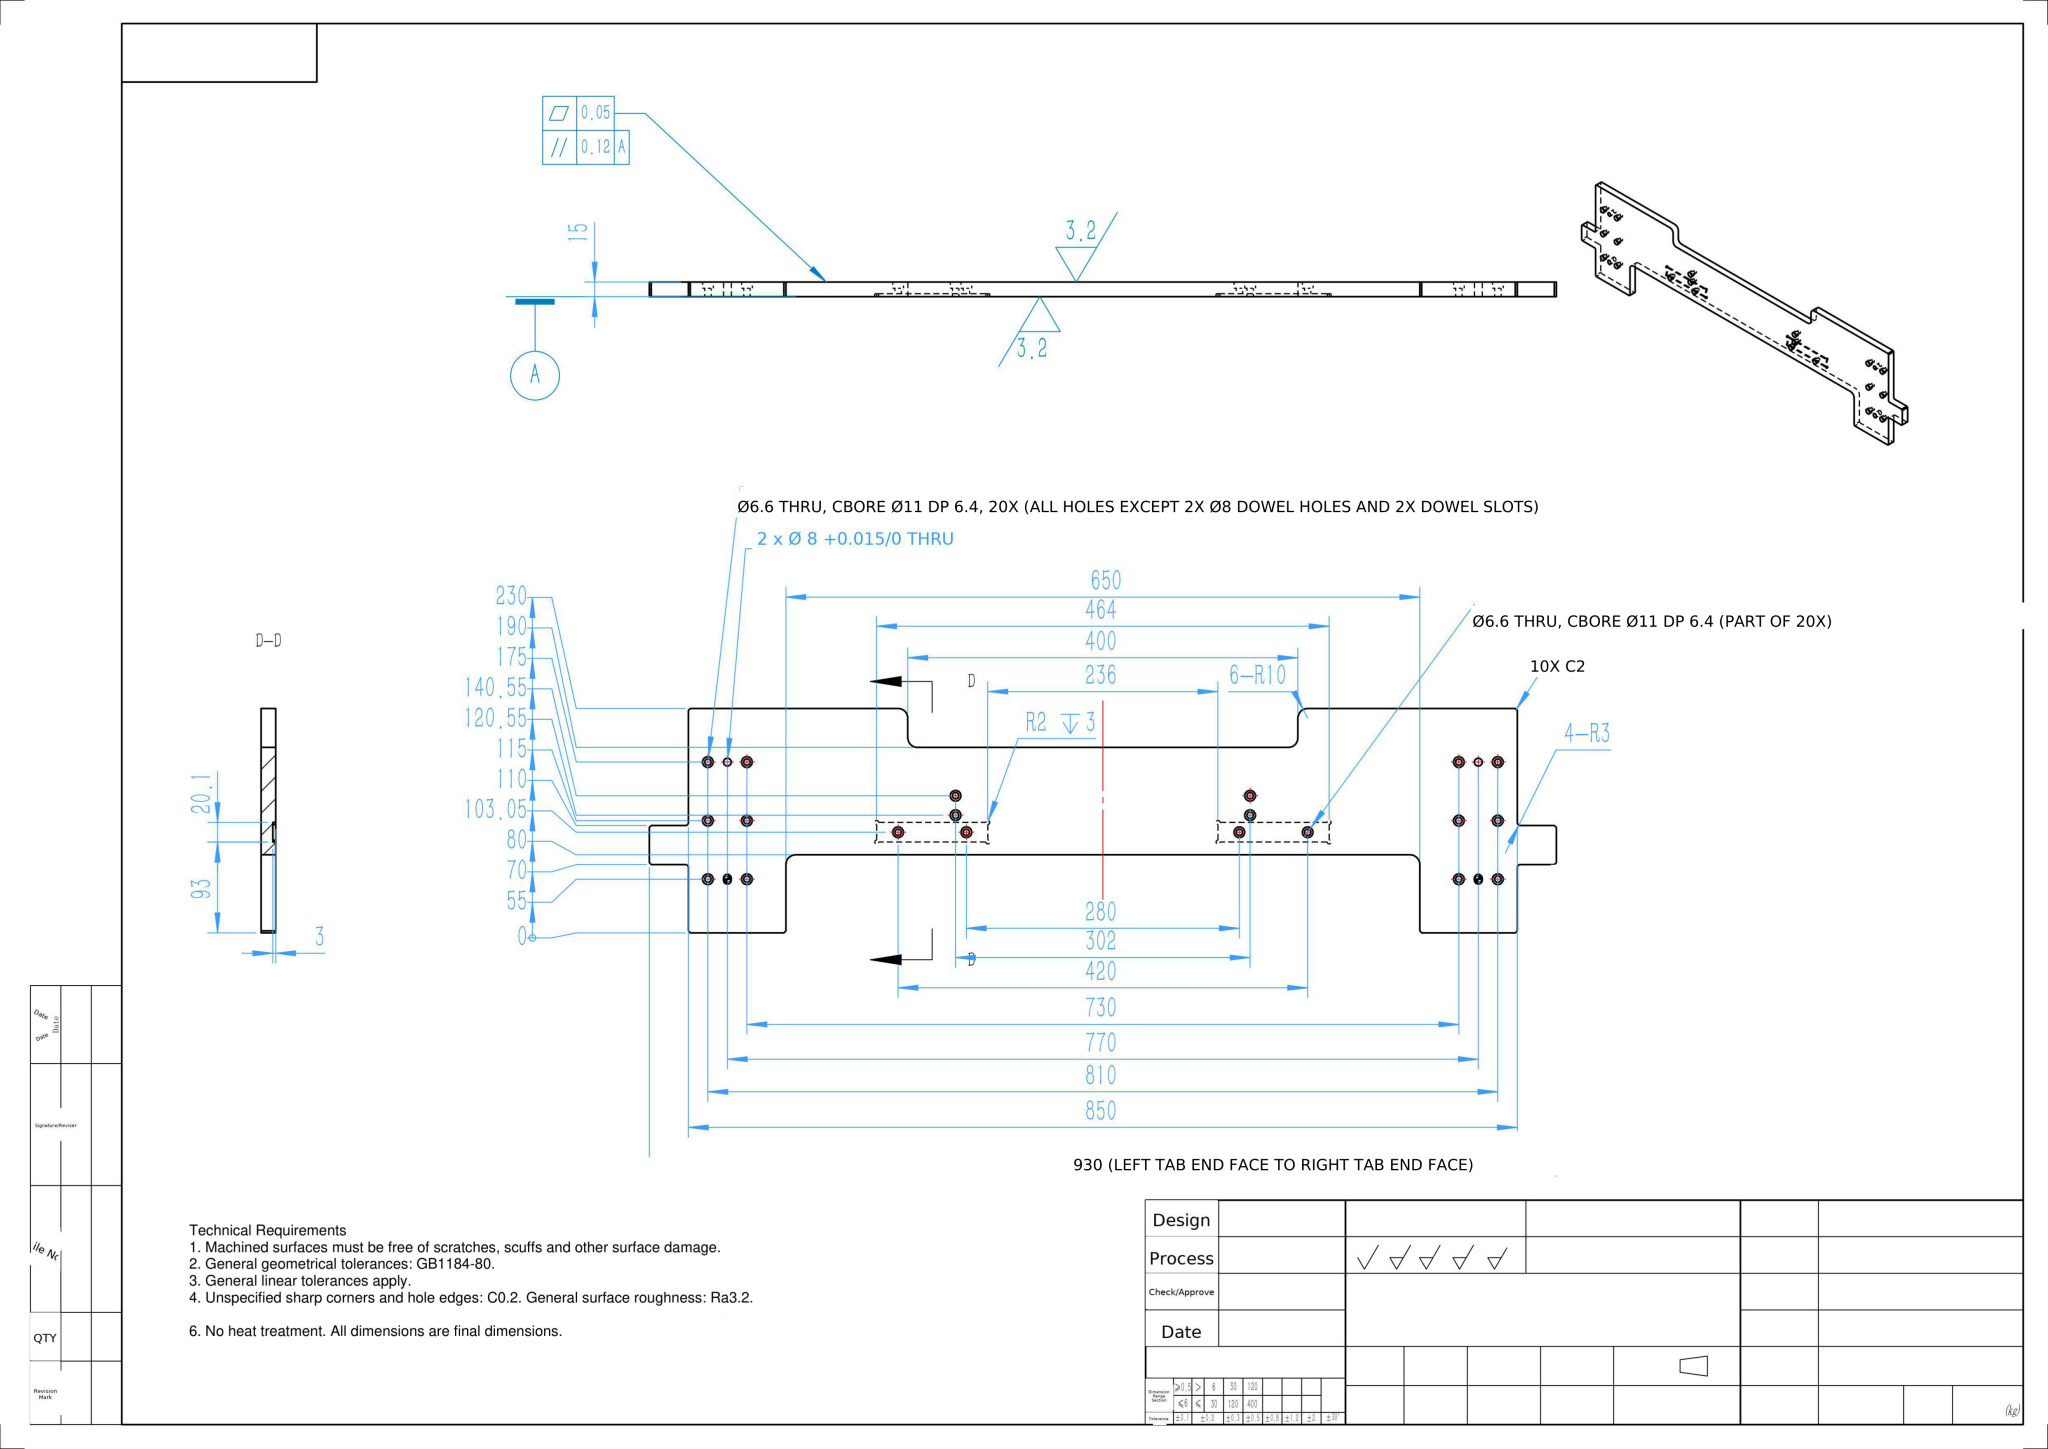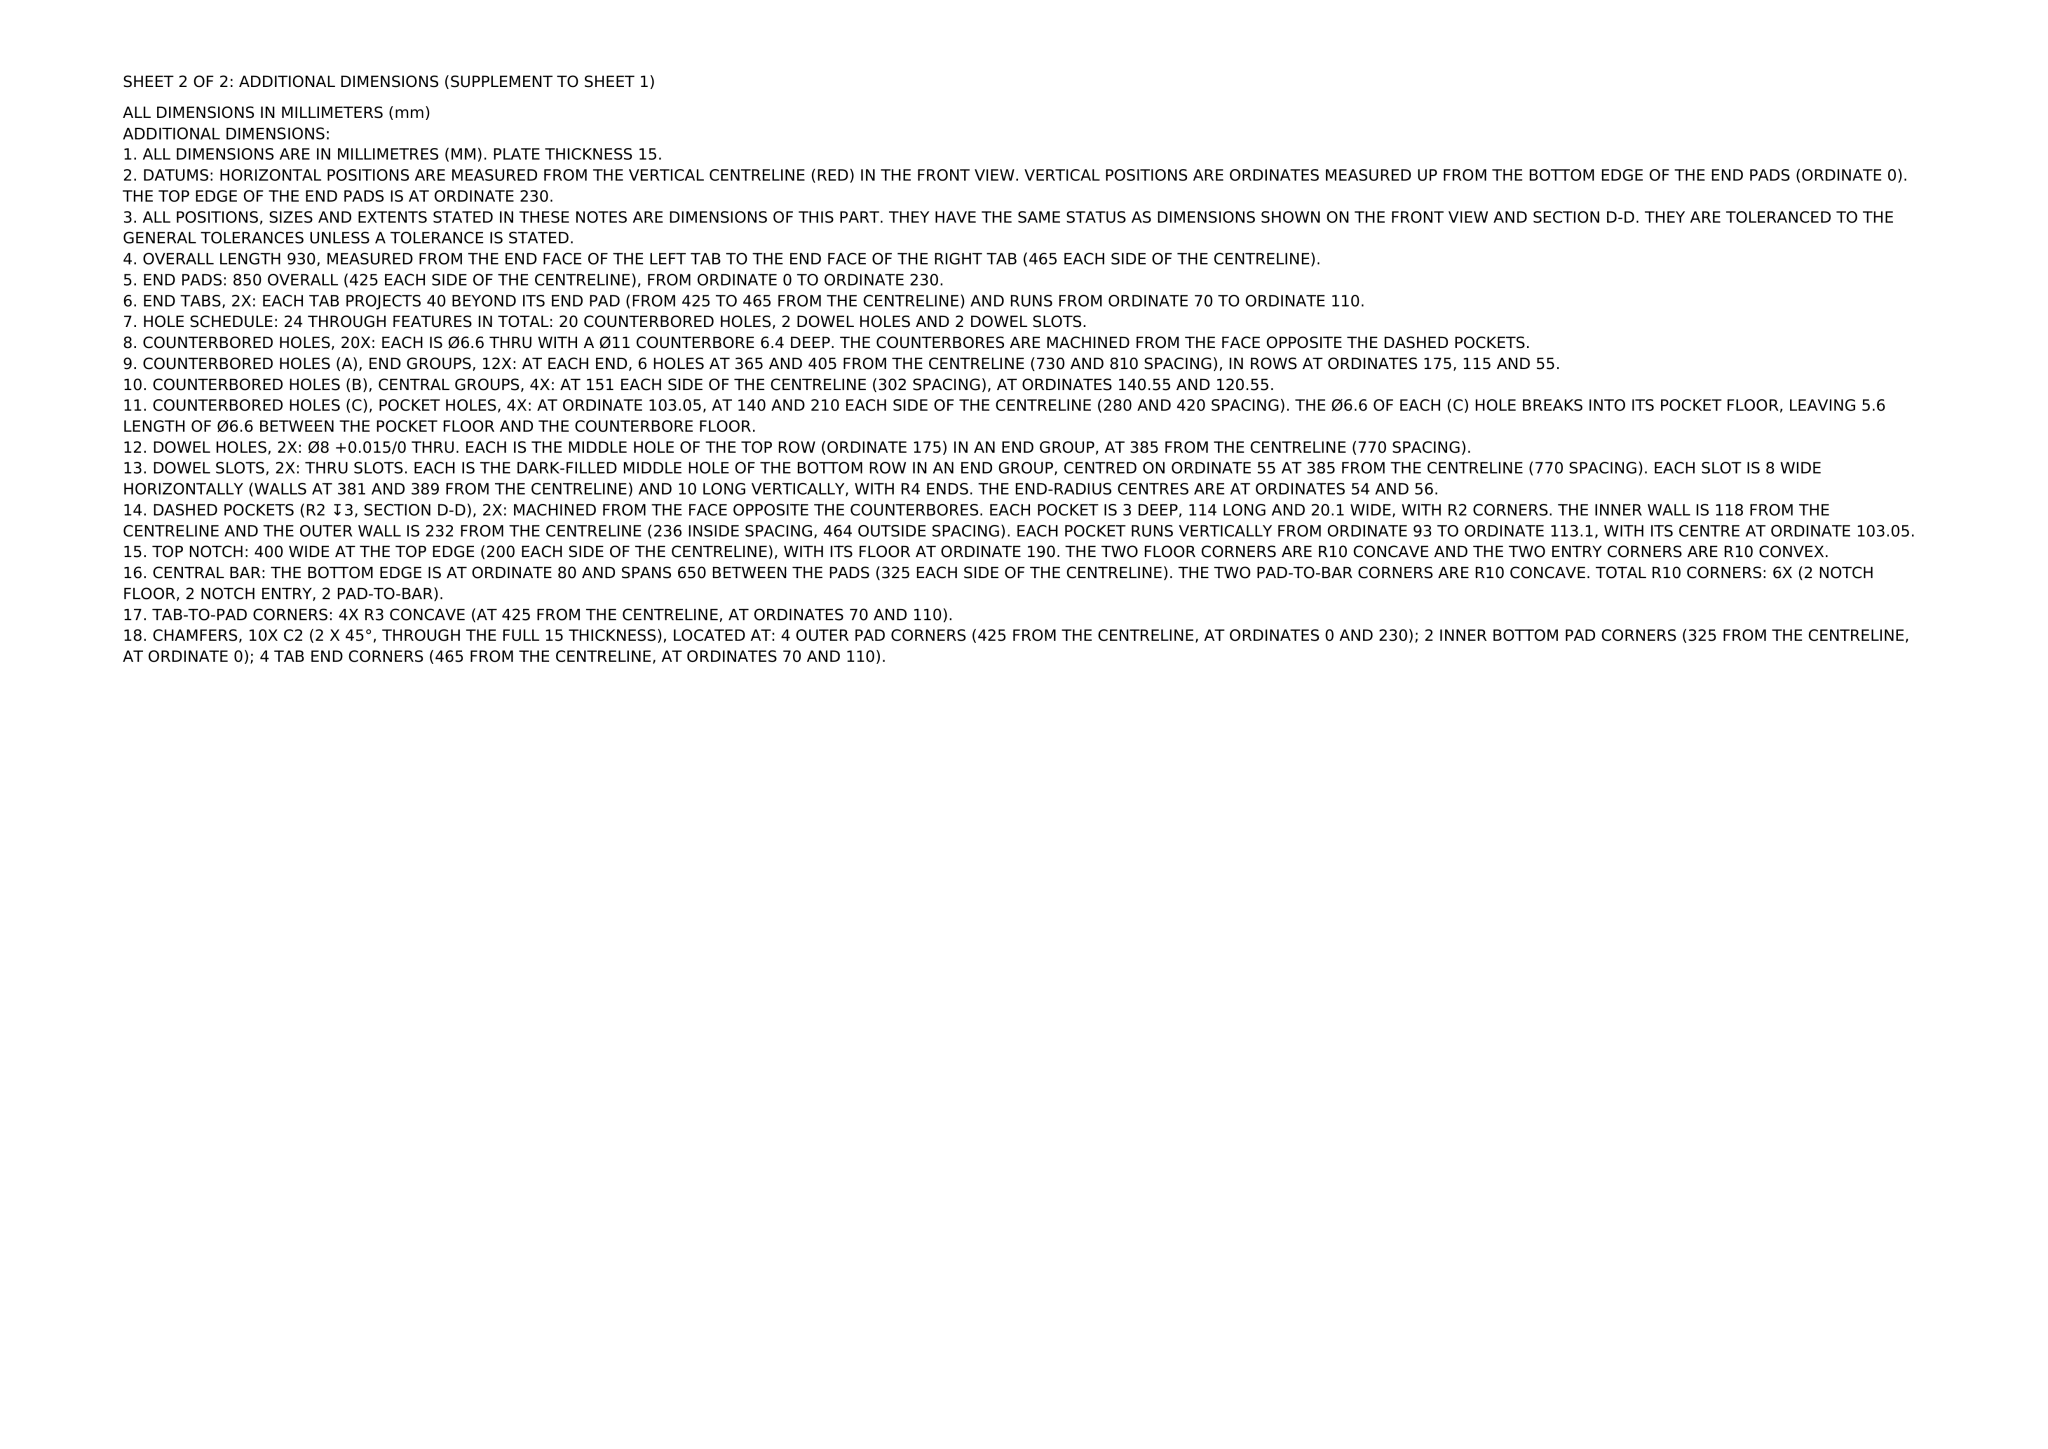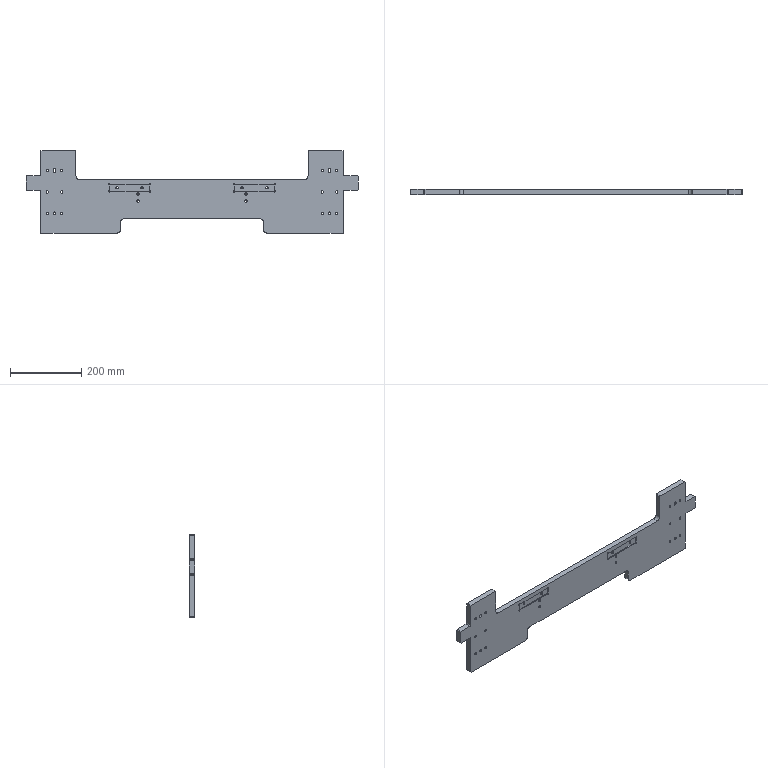Part | NX | mm | 1 solid | 178 faces | box 930 x 15 x 230 mm | volume 1925851 mm3 | cylinder 112 | plane 66 | commonest cylinder face diameters 11 x40 6.6 x40 4 x12 8 x10 20 x6 6 x4